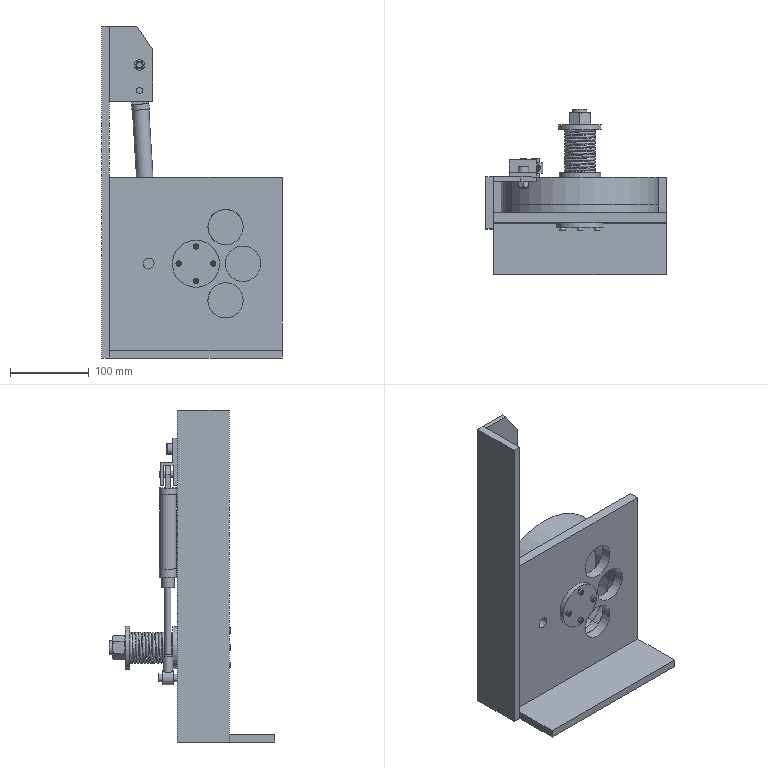Assembly | NX | mm | 20 component files | 36 solids | 359 faces | box 230 x 211 x 422.5 mm | volume 2483519 mm3 | plane 179 | cone 78 | cylinder 75 | torus 12 | sphere 10 | spline 5 | commonest cylinder face diameters 8 x12 4 x8 45 x7 25 x6 18 x4 3.838 x4 7 x4 10 x3
Bill of materials:
unnamed part 1 | 1 |  | Thin flat square plate with a pattern of circular through holes: one small hole, one medium central hole, and three large holes in an arc to one side, plus small holes in one edge face.
GB-T6170_F-2000,M8x1.25 | 1 |  | Hexagonal nut-like part: a hexagonal prism with a central circular through bore and chamfered corners on both faces.
GB-T70.1-2000,M8x20 | 1 |  | Hexagon Socket Head Cap Screw, GB-T 70.1-2000,M8x20
unnamed part 2 | 1 |  | Extruded bracket: a flat rectangular plate with two circular through holes, joined along one edge to an inverted U-shaped channel, giving an 'h'-shaped profile.
unnamed part 3 | 1 |  | Flanged cylindrical bushing: a cylindrical sleeve with a larger-diameter flange at one end and a central through bore.
unnamed part 4 | 1 |  | Plain solid cylindrical rod with flat ends.
unnamed part 5 | 1 |  | Thin L-shaped sheet bracket: a tall narrow vertical strip with a wider top tab that has two small holes and an angled corner, and a horizontal rectangular base flange at the bottom.
unnamed part 6 | 1 |  | Elongated telescopic cylinder-and-rod part: a larger cylindrical body, a slimmer rod coming out of one end, and a flat eyelet with a through hole at each end. It resembles a gas spring or damper.
unnamed part 7 | 1 |  | Short thin-walled cylindrical ring or tube section with a large central bore.
unnamed part 8 | 1 |  | Double-hub bushing: a central radial flange with a cylindrical hub on each side and a central through bore. The two hubs differ slightly in diameter and length.
unnamed part 9 | 1 |  | Flanged stepped shaft: a circular flange with four holes equally spaced on a circle, joined to a shaft with two diameters (a larger section next to the flange and a smaller section at the far end).
unnamed part 10 | 1 |  | Thin flat circular disc with a small central hole and an off-center kidney- or crescent-shaped through slot.
unnamed part 11 | 1 |  | Helical coil: many closely spaced turns of round-section wire forming an open cylindrical coil with a hollow center.
GB-T70.1-2000,M4x16 | 4 |  | Hexagon Socket Head Cap Screw, GB-T 70.1-2000,M4x16
unnamed part 12 | 1 |  | Flat circular disc with a central round through hole and one small cylindrical pin standing up from one face, set off-center.
GB-T6170_F-2000,M18x2.5 | 1 |  | Hexagonal prism with a central round bore. The outer corners are chamfered at both ends, which leaves curved edges on each flat face. This shape looks like a hex nut.
GB-T292_AC-1994,7005_AC | 1 |  | Annular assembly that looks like an open, single-row radial ball bearing: a concentric outer ring and inner ring, both with rectangular cross-sections, with a ring of spherical balls between them and a plain cylindrical bore through the middle.
Mates:
1. touch align | GB-T6170_F-2000_M18x2_5 1 face | spring_sleeve_2 1 face
2. touch align | GB-T6170_F-2000_M8x1_25 1 face | valve_body_mount 1 face